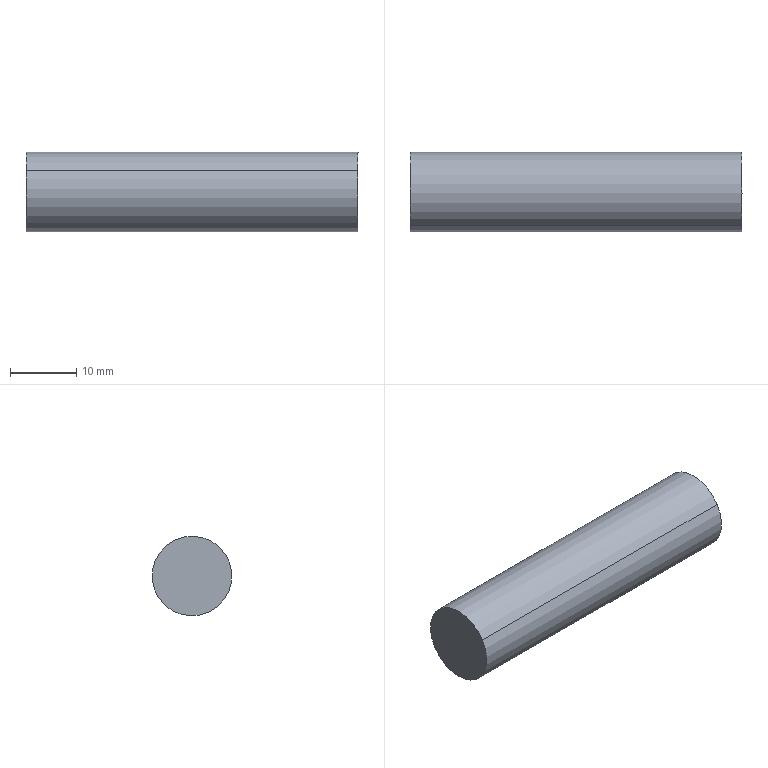Component | SolidWorks | Part1-1 | 1 solid | 4 faces | box 50 x 12 x 12 mm | volume 5655 mm3 | cylinder 2 | plane 2 | commonest cylinder face diameters 12 x2
build123d program:
from build123d import *

# Parameters (mm, degrees)
SKETCH1_R           = 6
BOSS_EXTRUDE1_DEPTH = 50


with BuildPart() as part:
    # Sketch1 → Boss-Extrude1 (new body)
    with BuildSketch(Plane.XY):
        Circle(SKETCH1_R)
    extrude(amount=BOSS_EXTRUDE1_DEPTH)


solid = part.part

# Placed as in the assembly
solid = solid.moved(Location((120.296, 56.837, 344.838), (0, 90, 0)))
STEP:
#1=COLOUR_RGB('',0.7922,0.8196,0.9333);
#2=FILL_AREA_STYLE_COLOUR('',#1);
#3=FILL_AREA_STYLE('',(#2));
#4=SURFACE_STYLE_FILL_AREA(#3);
#5=SURFACE_SIDE_STYLE('',(#4));
#6=SURFACE_STYLE_USAGE(.BOTH.,#5);
#7=PRESENTATION_STYLE_ASSIGNMENT((#6));
#8=CARTESIAN_POINT('',(6.705,2.039,13.704));
#9=VERTEX_POINT('',#8);
#10=CARTESIAN_POINT('',(6.705,2.437,13.449));
#11=VERTEX_POINT('',#10);
#12=CARTESIAN_POINT('',(6.705,2.238,13.576));
#13=DIRECTION('',(1.,0.,-0.));
#14=DIRECTION('',(0.,-0.8419,0.5397));
#15=AXIS2_PLACEMENT_3D('',#12,#13,#14);
#16=CIRCLE('',#15,0.2362);
#17=EDGE_CURVE('',#9,#11,#16,.T.);
#18=ORIENTED_EDGE('',*,*,#17,.F.);
#19=CARTESIAN_POINT('',(4.736,2.039,13.704));
#20=VERTEX_POINT('',#19);
#21=CARTESIAN_POINT('',(6.705,2.039,13.704));
#22=DIRECTION('',(-1.,-0.,0.));
#23=VECTOR('',#22,39.37);
#24=LINE('',#21,#23);
#25=EDGE_CURVE('',#9,#20,#24,.T.);
#26=ORIENTED_EDGE('',*,*,#25,.T.);
#27=CARTESIAN_POINT('',(4.736,2.437,13.449));
#28=VERTEX_POINT('',#27);
#29=CARTESIAN_POINT('',(4.736,2.238,13.576));
#30=DIRECTION('',(1.,0.,-0.));
#31=DIRECTION('',(0.,-0.8419,0.5397));
#32=AXIS2_PLACEMENT_3D('',#29,#30,#31);
#33=CIRCLE('',#32,0.2362);
#34=EDGE_CURVE('',#20,#28,#33,.T.);
#35=ORIENTED_EDGE('',*,*,#34,.T.);
#36=CARTESIAN_POINT('',(6.705,2.437,13.449));
#37=DIRECTION('',(-1.,-0.,0.));
#38=VECTOR('',#37,39.37);
#39=LINE('',#36,#38);
#40=EDGE_CURVE('',#11,#28,#39,.T.);
#41=ORIENTED_EDGE('',*,*,#40,.F.);
#42=EDGE_LOOP('',(#18,#26,#35,#41));
#43=FACE_OUTER_BOUND('',#42,.T.);
#44=CARTESIAN_POINT('',(6.705,2.238,13.576));
#45=DIRECTION('',(-1.,-0.,0.));
#46=DIRECTION('',(-0.,0.8419,-0.5397));
#47=AXIS2_PLACEMENT_3D('',#44,#45,#46);
#48=CYLINDRICAL_SURFACE('',#47,0.2362);
#49=ADVANCED_FACE('',(#43),#48,.T.);
#50=ORIENTED_EDGE('',*,*,#25,.F.);
#51=CARTESIAN_POINT('',(6.705,2.238,13.576));
#52=DIRECTION('',(1.,0.,-0.));
#53=DIRECTION('',(0.,-0.8419,0.5397));
#54=AXIS2_PLACEMENT_3D('',#51,#52,#53);
#55=CIRCLE('',#54,0.2362);
#56=EDGE_CURVE('',#11,#9,#55,.T.);
#57=ORIENTED_EDGE('',*,*,#56,.F.);
#58=ORIENTED_EDGE('',*,*,#40,.T.);
#59=CARTESIAN_POINT('',(4.736,2.238,13.576));
#60=DIRECTION('',(1.,0.,-0.));
#61=DIRECTION('',(0.,-0.8419,0.5397));
#62=AXIS2_PLACEMENT_3D('',#59,#60,#61);
#63=CIRCLE('',#62,0.2362);
#64=EDGE_CURVE('',#28,#20,#63,.T.);
#65=ORIENTED_EDGE('',*,*,#64,.T.);
#66=EDGE_LOOP('',(#50,#57,#58,#65));
#67=FACE_OUTER_BOUND('',#66,.T.);
#68=CARTESIAN_POINT('',(6.705,2.238,13.576));
#69=DIRECTION('',(-1.,-0.,0.));
#70=DIRECTION('',(-0.,0.8419,-0.5397));
#71=AXIS2_PLACEMENT_3D('',#68,#69,#70);
#72=CYLINDRICAL_SURFACE('',#71,0.2362);
#73=ADVANCED_FACE('',(#67),#72,.T.);
#74=ORIENTED_EDGE('',*,*,#56,.T.);
#75=ORIENTED_EDGE('',*,*,#17,.T.);
#76=EDGE_LOOP('',(#74,#75));
#77=FACE_OUTER_BOUND('',#76,.T.);
#78=CARTESIAN_POINT('',(6.705,2.238,13.576));
#79=DIRECTION('',(1.,0.,-0.));
#80=DIRECTION('',(0.,-0.8419,0.5397));
#81=AXIS2_PLACEMENT_3D('',#78,#79,#80);
#82=PLANE('',#81);
#83=ADVANCED_FACE('',(#77),#82,.T.);
#84=ORIENTED_EDGE('',*,*,#64,.F.);
#85=ORIENTED_EDGE('',*,*,#34,.F.);
#86=EDGE_LOOP('',(#84,#85));
#87=FACE_OUTER_BOUND('',#86,.T.);
#88=CARTESIAN_POINT('',(4.736,2.238,13.576));
#89=DIRECTION('',(1.,0.,-0.));
#90=DIRECTION('',(0.,-0.8419,0.5397));
#91=AXIS2_PLACEMENT_3D('',#88,#89,#90);
#92=PLANE('',#91);
#93=ADVANCED_FACE('',(#87),#92,.F.);
#94=CLOSED_SHELL('',(#49,#73,#83,#93));
#95=MANIFOLD_SOLID_BREP('',#94);
#96=STYLED_ITEM('',(#7),#95);
#97=(LENGTH_UNIT()NAMED_UNIT(*)SI_UNIT($,.METRE.));
#98=LENGTH_MEASURE_WITH_UNIT(LENGTH_MEASURE(0.0254),#97);
#99=DIMENSIONAL_EXPONENTS(1.,0.,0.,0.,0.,0.,0.);
#100=(CONVERSION_BASED_UNIT('',#98)LENGTH_UNIT()NAMED_UNIT(#99));
#101=UNCERTAINTY_MEASURE_WITH_UNIT(LENGTH_MEASURE(0.00001),#100,'','');
#102=(NAMED_UNIT(*)PLANE_ANGLE_UNIT()SI_UNIT($,.RADIAN.));
#103=(NAMED_UNIT(*)SI_UNIT($,.STERADIAN.)SOLID_ANGLE_UNIT());
#104=(GEOMETRIC_REPRESENTATION_CONTEXT(3)GLOBAL_UNCERTAINTY_ASSIGNED_CONTEXT((#101))GLOBAL_UNIT_ASSIGNED_CONTEXT((#100,#102,#103))REPRESENTATION_CONTEXT('',''));
#105=MECHANICAL_DESIGN_GEOMETRIC_PRESENTATION_REPRESENTATION('',(#96),#104);
#106=PRESENTATION_LAYER_ASSIGNMENT('','',(#96));
#107=CARTESIAN_POINT('',(0.,0.,0.));
#108=DIRECTION('',(0.,0.,1.));
#109=DIRECTION('',(1.,0.,0.));
#110=AXIS2_PLACEMENT_3D('',#107,#108,#109);
#111=(LENGTH_UNIT()NAMED_UNIT(*)SI_UNIT($,.METRE.));
#112=LENGTH_MEASURE_WITH_UNIT(LENGTH_MEASURE(0.0254),#111);
#113=DIMENSIONAL_EXPONENTS(1.,0.,0.,0.,0.,0.,0.);
#114=(CONVERSION_BASED_UNIT('',#112)LENGTH_UNIT()NAMED_UNIT(#113));
#115=UNCERTAINTY_MEASURE_WITH_UNIT(LENGTH_MEASURE(0.00001),#114,'','');
#116=(NAMED_UNIT(*)PLANE_ANGLE_UNIT()SI_UNIT($,.RADIAN.));
#117=(NAMED_UNIT(*)SI_UNIT($,.STERADIAN.)SOLID_ANGLE_UNIT());
#118=(GEOMETRIC_REPRESENTATION_CONTEXT(3)GLOBAL_UNCERTAINTY_ASSIGNED_CONTEXT((#115))GLOBAL_UNIT_ASSIGNED_CONTEXT((#114,#116,#117))REPRESENTATION_CONTEXT('',''));
#119=ADVANCED_BREP_SHAPE_REPRESENTATION('',(#95,#110),#118);